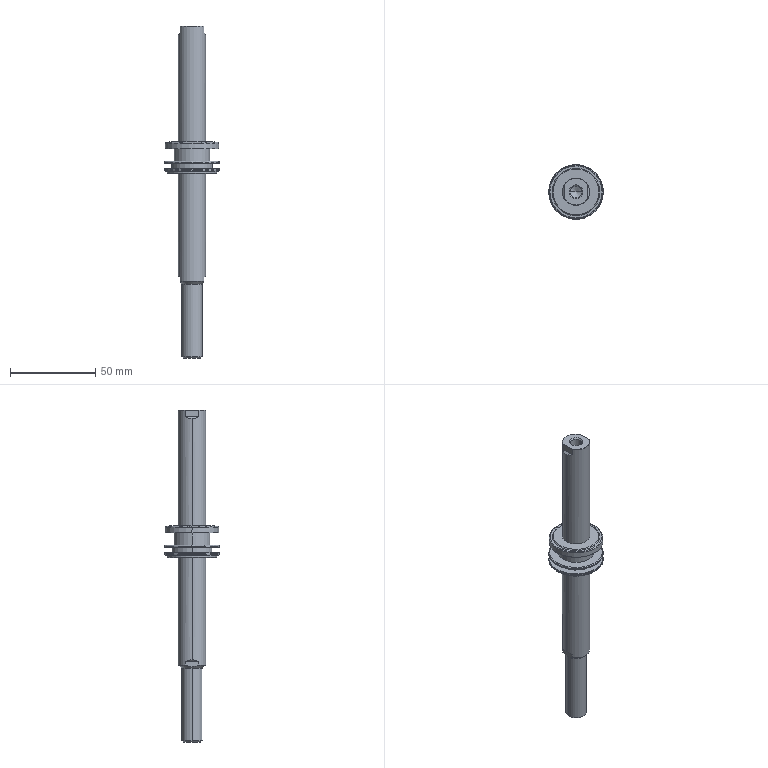Component | SolidWorks | JDAD32x50-20-SE2-1_GAN-1 | 1 solid | 64 faces | volume 41057 mm3 | cylinder 20 | plane 18 | cone 16 | spline 10 | commonest cylinder face diameters 16 x4 32 x4 6.647 x2 31.6 x2 20.8 x2 24 x2 29 x2 12 x2